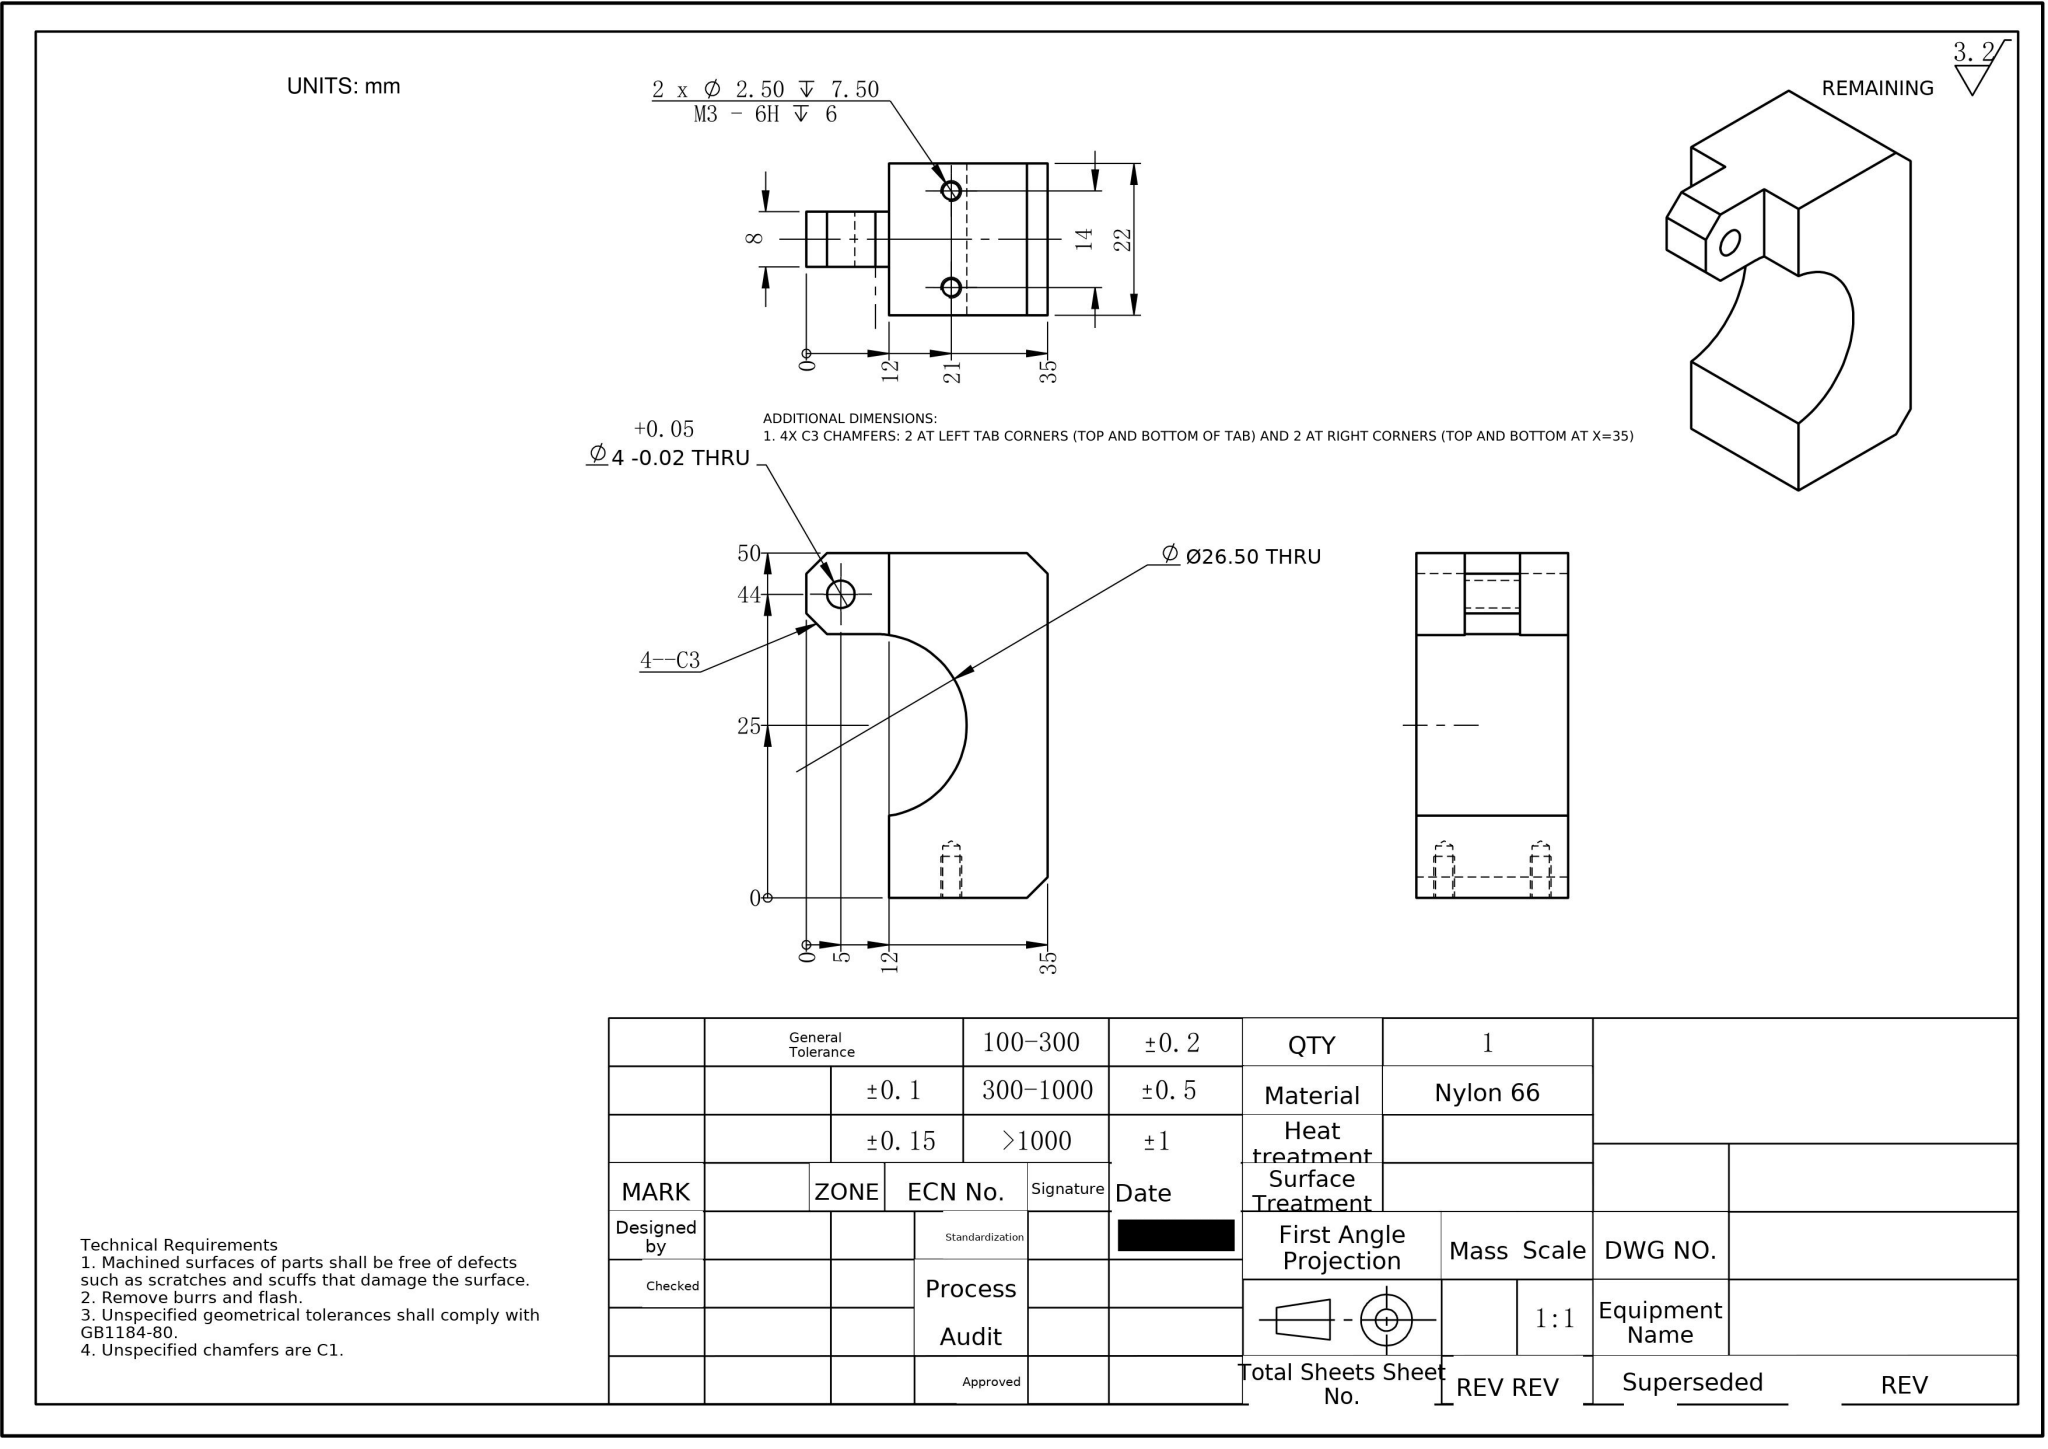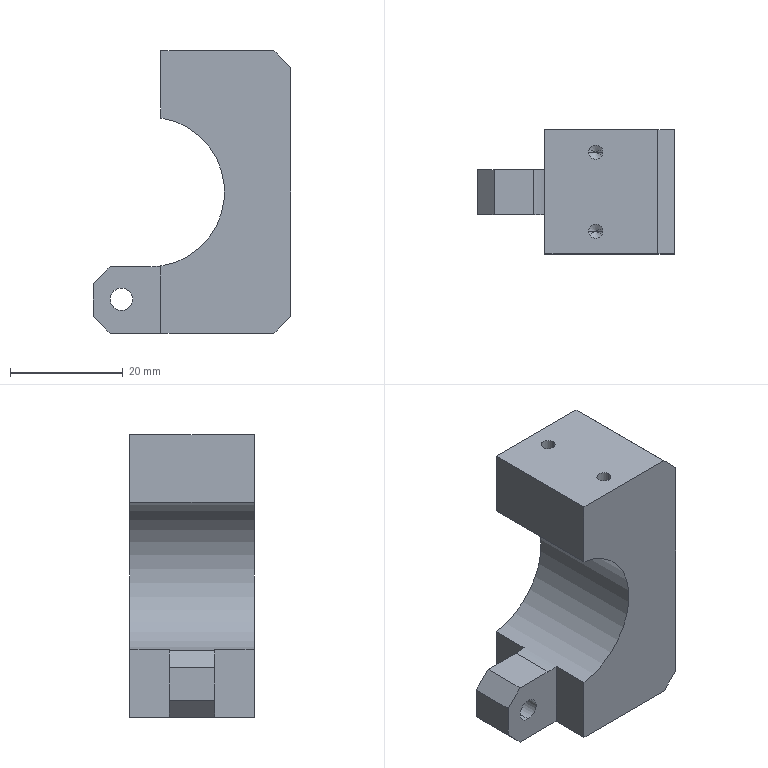Part | NX | mm | 1 solid | 27 faces | box 35 x 22 x 50 mm | volume 21077 mm3 | plane 16 | cylinder 7 | cone 4 | commonest cylinder face diameters 2.5 x4 4 x2 26.5 x1
STEP:
#1=COLOUR_RGB('',0.7922,0.8196,0.9333);
#2=FILL_AREA_STYLE_COLOUR('',#1);
#3=FILL_AREA_STYLE('',(#2));
#4=SURFACE_STYLE_FILL_AREA(#3);
#5=SURFACE_SIDE_STYLE('',(#4));
#6=SURFACE_STYLE_USAGE(.BOTH.,#5);
#7=PRESENTATION_STYLE_ASSIGNMENT((#6));
#8=CARTESIAN_POINT('',(-2.75,-7.,17.5));
#9=VERTEX_POINT('',#8);
#10=CARTESIAN_POINT('',(-0.25,-7.,17.5));
#11=VERTEX_POINT('',#10);
#12=CARTESIAN_POINT('',(-1.5,-7.,17.5));
#13=DIRECTION('',(0.,0.,1.));
#14=DIRECTION('',(1.,0.,0.));
#15=AXIS2_PLACEMENT_3D('',#12,#13,#14);
#16=CIRCLE('',#15,1.25);
#17=EDGE_CURVE('',#9,#11,#16,.T.);
#18=ORIENTED_EDGE('',*,*,#17,.F.);
#19=CARTESIAN_POINT('',(-2.75,-7.,25.));
#20=VERTEX_POINT('',#19);
#21=CARTESIAN_POINT('',(-2.75,-7.,25.));
#22=DIRECTION('',(0.,0.,1.));
#23=VECTOR('',#22,1000.);
#24=LINE('',#21,#23);
#25=EDGE_CURVE('',#9,#20,#24,.T.);
#26=ORIENTED_EDGE('',*,*,#25,.T.);
#27=CARTESIAN_POINT('',(-0.25,-7.,25.));
#28=VERTEX_POINT('',#27);
#29=CARTESIAN_POINT('',(-1.5,-7.,25.));
#30=DIRECTION('',(0.,0.,1.));
#31=DIRECTION('',(1.,0.,0.));
#32=AXIS2_PLACEMENT_3D('',#29,#30,#31);
#33=CIRCLE('',#32,1.25);
#34=EDGE_CURVE('',#20,#28,#33,.T.);
#35=ORIENTED_EDGE('',*,*,#34,.T.);
#36=CARTESIAN_POINT('',(-0.25,-7.,25.));
#37=DIRECTION('',(0.,0.,1.));
#38=VECTOR('',#37,1000.);
#39=LINE('',#36,#38);
#40=EDGE_CURVE('',#11,#28,#39,.T.);
#41=ORIENTED_EDGE('',*,*,#40,.F.);
#42=EDGE_LOOP('',(#18,#26,#35,#41));
#43=FACE_OUTER_BOUND('',#42,.T.);
#44=CARTESIAN_POINT('',(-1.5,-7.,25.));
#45=DIRECTION('',(0.,0.,1.));
#46=DIRECTION('',(1.,0.,0.));
#47=AXIS2_PLACEMENT_3D('',#44,#45,#46);
#48=CYLINDRICAL_SURFACE('',#47,1.25);
#49=ADVANCED_FACE('',(#43),#48,.F.);
#50=CARTESIAN_POINT('',(-1.5,-7.,16.749));
#51=VERTEX_POINT('',#50);
#52=CARTESIAN_POINT('',(-0.25,-7.,17.5));
#53=DIRECTION('',(0.8572,0.,0.515));
#54=VECTOR('',#53,1000.);
#55=LINE('',#52,#54);
#56=EDGE_CURVE('',#51,#11,#55,.T.);
#57=ORIENTED_EDGE('',*,*,#56,.F.);
#58=CARTESIAN_POINT('',(-2.75,-7.,17.5));
#59=DIRECTION('',(-0.8572,0.,0.515));
#60=VECTOR('',#59,1000.);
#61=LINE('',#58,#60);
#62=EDGE_CURVE('',#51,#9,#61,.T.);
#63=ORIENTED_EDGE('',*,*,#62,.T.);
#64=ORIENTED_EDGE('',*,*,#17,.T.);
#65=EDGE_LOOP('',(#57,#63,#64));
#66=FACE_OUTER_BOUND('',#65,.T.);
#67=CARTESIAN_POINT('',(-1.5,-7.,17.5));
#68=DIRECTION('',(0.,0.,1.));
#69=DIRECTION('',(1.,0.,0.));
#70=AXIS2_PLACEMENT_3D('',#67,#68,#69);
#71=CONICAL_SURFACE('',#70,1.25,1.03);
#72=ADVANCED_FACE('',(#66),#71,.F.);
#73=CARTESIAN_POINT('',(-2.75,7.,17.5));
#74=VERTEX_POINT('',#73);
#75=CARTESIAN_POINT('',(-0.25,7.,17.5));
#76=VERTEX_POINT('',#75);
#77=CARTESIAN_POINT('',(-1.5,7.,17.5));
#78=DIRECTION('',(0.,0.,1.));
#79=DIRECTION('',(1.,0.,0.));
#80=AXIS2_PLACEMENT_3D('',#77,#78,#79);
#81=CIRCLE('',#80,1.25);
#82=EDGE_CURVE('',#74,#76,#81,.T.);
#83=ORIENTED_EDGE('',*,*,#82,.F.);
#84=CARTESIAN_POINT('',(-2.75,7.,25.));
#85=VERTEX_POINT('',#84);
#86=CARTESIAN_POINT('',(-2.75,7.,25.));
#87=DIRECTION('',(0.,0.,1.));
#88=VECTOR('',#87,1000.);
#89=LINE('',#86,#88);
#90=EDGE_CURVE('',#74,#85,#89,.T.);
#91=ORIENTED_EDGE('',*,*,#90,.T.);
#92=CARTESIAN_POINT('',(-0.25,7.,25.));
#93=VERTEX_POINT('',#92);
#94=CARTESIAN_POINT('',(-1.5,7.,25.));
#95=DIRECTION('',(0.,0.,1.));
#96=DIRECTION('',(1.,0.,0.));
#97=AXIS2_PLACEMENT_3D('',#94,#95,#96);
#98=CIRCLE('',#97,1.25);
#99=EDGE_CURVE('',#85,#93,#98,.T.);
#100=ORIENTED_EDGE('',*,*,#99,.T.);
#101=CARTESIAN_POINT('',(-0.25,7.,25.));
#102=DIRECTION('',(0.,0.,1.));
#103=VECTOR('',#102,1000.);
#104=LINE('',#101,#103);
#105=EDGE_CURVE('',#76,#93,#104,.T.);
#106=ORIENTED_EDGE('',*,*,#105,.F.);
#107=EDGE_LOOP('',(#83,#91,#100,#106));
#108=FACE_OUTER_BOUND('',#107,.T.);
#109=CARTESIAN_POINT('',(-1.5,7.,25.));
#110=DIRECTION('',(0.,0.,1.));
#111=DIRECTION('',(1.,0.,0.));
#112=AXIS2_PLACEMENT_3D('',#109,#110,#111);
#113=CYLINDRICAL_SURFACE('',#112,1.25);
#114=ADVANCED_FACE('',(#108),#113,.F.);
#115=CARTESIAN_POINT('',(-1.5,7.,16.749));
#116=VERTEX_POINT('',#115);
#117=CARTESIAN_POINT('',(-0.25,7.,17.5));
#118=DIRECTION('',(0.8572,0.,0.515));
#119=VECTOR('',#118,1000.);
#120=LINE('',#117,#119);
#121=EDGE_CURVE('',#116,#76,#120,.T.);
#122=ORIENTED_EDGE('',*,*,#121,.F.);
#123=CARTESIAN_POINT('',(-2.75,7.,17.5));
#124=DIRECTION('',(-0.8572,0.,0.515));
#125=VECTOR('',#124,1000.);
#126=LINE('',#123,#125);
#127=EDGE_CURVE('',#116,#74,#126,.T.);
#128=ORIENTED_EDGE('',*,*,#127,.T.);
#129=ORIENTED_EDGE('',*,*,#82,.T.);
#130=EDGE_LOOP('',(#122,#128,#129));
#131=FACE_OUTER_BOUND('',#130,.T.);
#132=CARTESIAN_POINT('',(-1.5,7.,17.5));
#133=DIRECTION('',(0.,0.,1.));
#134=DIRECTION('',(1.,0.,0.));
#135=AXIS2_PLACEMENT_3D('',#132,#133,#134);
#136=CONICAL_SURFACE('',#135,1.25,1.03);
#137=ADVANCED_FACE('',(#131),#136,.F.);
#138=CARTESIAN_POINT('',(-17.5,4.,-17.));
#139=VERTEX_POINT('',#138);
#140=CARTESIAN_POINT('',(-17.5,4.,-21.));
#141=VERTEX_POINT('',#140);
#142=CARTESIAN_POINT('',(-17.5,4.,-19.));
#143=DIRECTION('',(0.,-1.,0.));
#144=DIRECTION('',(0.,0.,-1.));
#145=AXIS2_PLACEMENT_3D('',#142,#143,#144);
#146=CIRCLE('',#145,2.);
#147=EDGE_CURVE('',#139,#141,#146,.T.);
#148=ORIENTED_EDGE('',*,*,#147,.F.);
#149=CARTESIAN_POINT('',(-17.5,-4.,-17.));
#150=VERTEX_POINT('',#149);
#151=CARTESIAN_POINT('',(-17.5,6.,-17.));
#152=DIRECTION('',(0.,-1.,0.));
#153=VECTOR('',#152,1000.);
#154=LINE('',#151,#153);
#155=EDGE_CURVE('',#139,#150,#154,.T.);
#156=ORIENTED_EDGE('',*,*,#155,.T.);
#157=CARTESIAN_POINT('',(-17.5,-4.,-21.));
#158=VERTEX_POINT('',#157);
#159=CARTESIAN_POINT('',(-17.5,-4.,-19.));
#160=DIRECTION('',(0.,-1.,0.));
#161=DIRECTION('',(0.,0.,-1.));
#162=AXIS2_PLACEMENT_3D('',#159,#160,#161);
#163=CIRCLE('',#162,2.);
#164=EDGE_CURVE('',#150,#158,#163,.T.);
#165=ORIENTED_EDGE('',*,*,#164,.T.);
#166=CARTESIAN_POINT('',(-17.5,6.,-21.));
#167=DIRECTION('',(0.,-1.,0.));
#168=VECTOR('',#167,1000.);
#169=LINE('',#166,#168);
#170=EDGE_CURVE('',#141,#158,#169,.T.);
#171=ORIENTED_EDGE('',*,*,#170,.F.);
#172=EDGE_LOOP('',(#148,#156,#165,#171));
#173=FACE_OUTER_BOUND('',#172,.T.);
#174=CARTESIAN_POINT('',(-17.5,6.,-19.));
#175=DIRECTION('',(0.,-1.,0.));
#176=DIRECTION('',(0.,0.,-1.));
#177=AXIS2_PLACEMENT_3D('',#174,#175,#176);
#178=CYLINDRICAL_SURFACE('',#177,2.);
#179=ADVANCED_FACE('',(#173),#178,.F.);
#180=CARTESIAN_POINT('',(12.5,11.,22.));
#181=VERTEX_POINT('',#180);
#182=CARTESIAN_POINT('',(12.5,11.,-22.));
#183=VERTEX_POINT('',#182);
#184=CARTESIAN_POINT('',(12.5,11.,25.));
#185=DIRECTION('',(0.,0.,-1.));
#186=VECTOR('',#185,1000.);
#187=LINE('',#184,#186);
#188=EDGE_CURVE('',#181,#183,#187,.T.);
#189=ORIENTED_EDGE('',*,*,#188,.F.);
#190=CARTESIAN_POINT('',(12.5,-11.,22.));
#191=VERTEX_POINT('',#190);
#192=CARTESIAN_POINT('',(12.5,11.,22.));
#193=DIRECTION('',(0.,-1.,0.));
#194=VECTOR('',#193,1000.);
#195=LINE('',#192,#194);
#196=EDGE_CURVE('',#181,#191,#195,.T.);
#197=ORIENTED_EDGE('',*,*,#196,.T.);
#198=CARTESIAN_POINT('',(12.5,-11.,-22.));
#199=VERTEX_POINT('',#198);
#200=CARTESIAN_POINT('',(12.5,-11.,25.));
#201=DIRECTION('',(0.,0.,-1.));
#202=VECTOR('',#201,1000.);
#203=LINE('',#200,#202);
#204=EDGE_CURVE('',#191,#199,#203,.T.);
#205=ORIENTED_EDGE('',*,*,#204,.T.);
#206=CARTESIAN_POINT('',(12.5,11.,-22.));
#207=DIRECTION('',(0.,1.,0.));
#208=VECTOR('',#207,1000.);
#209=LINE('',#206,#208);
#210=EDGE_CURVE('',#199,#183,#209,.T.);
#211=ORIENTED_EDGE('',*,*,#210,.T.);
#212=EDGE_LOOP('',(#189,#197,#205,#211));
#213=FACE_OUTER_BOUND('',#212,.T.);
#214=CARTESIAN_POINT('',(12.5,11.,25.));
#215=DIRECTION('',(-1.,0.,0.));
#216=DIRECTION('',(0.,0.,1.));
#217=AXIS2_PLACEMENT_3D('',#214,#215,#216);
#218=PLANE('',#217);
#219=ADVANCED_FACE('',(#213),#218,.F.);
#220=CARTESIAN_POINT('',(-10.5,-4.,-25.));
#221=VERTEX_POINT('',#220);
#222=CARTESIAN_POINT('',(-10.5,-11.,-25.));
#223=VERTEX_POINT('',#222);
#224=CARTESIAN_POINT('',(-10.5,-4.,-25.));
#225=DIRECTION('',(0.,-1.,0.));
#226=VECTOR('',#225,1000.);
#227=LINE('',#224,#226);
#228=EDGE_CURVE('',#221,#223,#227,.T.);
#229=ORIENTED_EDGE('',*,*,#228,.F.);
#230=CARTESIAN_POINT('',(-19.5,-4.,-25.));
#231=VERTEX_POINT('',#230);
#232=CARTESIAN_POINT('',(-22.5,-4.,-25.));
#233=DIRECTION('',(1.,0.,0.));
#234=VECTOR('',#233,1000.);
#235=LINE('',#232,#234);
#236=EDGE_CURVE('',#231,#221,#235,.T.);
#237=ORIENTED_EDGE('',*,*,#236,.F.);
#238=CARTESIAN_POINT('',(-19.5,4.,-25.));
#239=VERTEX_POINT('',#238);
#240=CARTESIAN_POINT('',(-19.5,11.,-25.));
#241=DIRECTION('',(0.,1.,0.));
#242=VECTOR('',#241,1000.);
#243=LINE('',#240,#242);
#244=EDGE_CURVE('',#231,#239,#243,.T.);
#245=ORIENTED_EDGE('',*,*,#244,.T.);
#246=CARTESIAN_POINT('',(-10.5,4.,-25.));
#247=VERTEX_POINT('',#246);
#248=CARTESIAN_POINT('',(-22.5,4.,-25.));
#249=DIRECTION('',(1.,0.,0.));
#250=VECTOR('',#249,1000.);
#251=LINE('',#248,#250);
#252=EDGE_CURVE('',#239,#247,#251,.T.);
#253=ORIENTED_EDGE('',*,*,#252,.T.);
#254=CARTESIAN_POINT('',(-10.5,11.,-25.));
#255=VERTEX_POINT('',#254);
#256=CARTESIAN_POINT('',(-10.5,4.,-25.));
#257=DIRECTION('',(0.,-1.,0.));
#258=VECTOR('',#257,1000.);
#259=LINE('',#256,#258);
#260=EDGE_CURVE('',#255,#247,#259,.T.);
#261=ORIENTED_EDGE('',*,*,#260,.F.);
#262=CARTESIAN_POINT('',(9.5,11.,-25.));
#263=VERTEX_POINT('',#262);
#264=CARTESIAN_POINT('',(-12.5,11.,-25.));
#265=DIRECTION('',(-1.,0.,0.));
#266=VECTOR('',#265,1000.);
#267=LINE('',#264,#266);
#268=EDGE_CURVE('',#263,#255,#267,.T.);
#269=ORIENTED_EDGE('',*,*,#268,.F.);
#270=CARTESIAN_POINT('',(9.5,-11.,-25.));
#271=VERTEX_POINT('',#270);
#272=CARTESIAN_POINT('',(9.5,11.,-25.));
#273=DIRECTION('',(0.,-1.,0.));
#274=VECTOR('',#273,1000.);
#275=LINE('',#272,#274);
#276=EDGE_CURVE('',#263,#271,#275,.T.);
#277=ORIENTED_EDGE('',*,*,#276,.T.);
#278=CARTESIAN_POINT('',(-12.5,-11.,-25.));
#279=DIRECTION('',(-1.,0.,0.));
#280=VECTOR('',#279,1000.);
#281=LINE('',#278,#280);
#282=EDGE_CURVE('',#271,#223,#281,.T.);
#283=ORIENTED_EDGE('',*,*,#282,.T.);
#284=EDGE_LOOP('',(#229,#237,#245,#253,#261,#269,#277,#283));
#285=FACE_OUTER_BOUND('',#284,.T.);
#286=CARTESIAN_POINT('',(-12.5,11.,-25.));
#287=DIRECTION('',(0.,0.,1.));
#288=DIRECTION('',(1.,0.,0.));
#289=AXIS2_PLACEMENT_3D('',#286,#287,#288);
#290=PLANE('',#289);
#291=ADVANCED_FACE('',(#285),#290,.F.);
#292=CARTESIAN_POINT('',(-1.5,-7.,25.));
#293=DIRECTION('',(0.,0.,1.));
#294=DIRECTION('',(1.,0.,0.));
#295=AXIS2_PLACEMENT_3D('',#292,#293,#294);
#296=CIRCLE('',#295,1.25);
#297=EDGE_CURVE('',#28,#20,#296,.T.);
#298=ORIENTED_EDGE('',*,*,#297,.F.);
#299=ORIENTED_EDGE('',*,*,#34,.F.);
#300=EDGE_LOOP('',(#298,#299));
#301=FACE_BOUND('',#300,.T.);
#302=CARTESIAN_POINT('',(-1.5,7.,25.));
#303=DIRECTION('',(0.,0.,1.));
#304=DIRECTION('',(1.,0.,0.));
#305=AXIS2_PLACEMENT_3D('',#302,#303,#304);
#306=CIRCLE('',#305,1.25);
#307=EDGE_CURVE('',#93,#85,#306,.T.);
#308=ORIENTED_EDGE('',*,*,#307,.F.);
#309=ORIENTED_EDGE('',*,*,#99,.F.);
#310=EDGE_LOOP('',(#308,#309));
#311=FACE_BOUND('',#310,.T.);
#312=CARTESIAN_POINT('',(-10.5,11.,25.));
#313=VERTEX_POINT('',#312);
#314=CARTESIAN_POINT('',(9.5,11.,25.));
#315=VERTEX_POINT('',#314);
#316=CARTESIAN_POINT('',(-12.5,11.,25.));
#317=DIRECTION('',(1.,0.,0.));
#318=VECTOR('',#317,1000.);
#319=LINE('',#316,#318);
#320=EDGE_CURVE('',#313,#315,#319,.T.);
#321=ORIENTED_EDGE('',*,*,#320,.F.);
#322=CARTESIAN_POINT('',(-10.5,-11.,25.));
#323=VERTEX_POINT('',#322);
#324=CARTESIAN_POINT('',(-10.5,39.,25.));
#325=DIRECTION('',(0.,-1.,0.));
#326=VECTOR('',#325,1000.);
#327=LINE('',#324,#326);
#328=EDGE_CURVE('',#313,#323,#327,.T.);
#329=ORIENTED_EDGE('',*,*,#328,.T.);
#330=CARTESIAN_POINT('',(9.5,-11.,25.));
#331=VERTEX_POINT('',#330);
#332=CARTESIAN_POINT('',(-12.5,-11.,25.));
#333=DIRECTION('',(1.,0.,0.));
#334=VECTOR('',#333,1000.);
#335=LINE('',#332,#334);
#336=EDGE_CURVE('',#323,#331,#335,.T.);
#337=ORIENTED_EDGE('',*,*,#336,.T.);
#338=CARTESIAN_POINT('',(9.5,11.,25.));
#339=DIRECTION('',(0.,1.,0.));
#340=VECTOR('',#339,1000.);
#341=LINE('',#338,#340);
#342=EDGE_CURVE('',#331,#315,#341,.T.);
#343=ORIENTED_EDGE('',*,*,#342,.T.);
#344=EDGE_LOOP('',(#321,#329,#337,#343));
#345=FACE_OUTER_BOUND('',#344,.T.);
#346=CARTESIAN_POINT('',(-12.5,11.,25.));
#347=DIRECTION('',(0.,0.,-1.));
#348=DIRECTION('',(-1.,0.,0.));
#349=AXIS2_PLACEMENT_3D('',#346,#347,#348);
#350=PLANE('',#349);
#351=ADVANCED_FACE('',(#301,#311,#345),#350,.F.);
#352=ORIENTED_EDGE('',*,*,#268,.T.);
#353=CARTESIAN_POINT('',(-10.5,11.,-13.098));
#354=VERTEX_POINT('',#353);
#355=CARTESIAN_POINT('',(-10.5,11.,-5.));
#356=DIRECTION('',(0.,0.,-1.));
#357=VECTOR('',#356,1000.);
#358=LINE('',#355,#357);
#359=EDGE_CURVE('',#354,#255,#358,.T.);
#360=ORIENTED_EDGE('',*,*,#359,.F.);
#361=CARTESIAN_POINT('',(-10.5,11.,13.098));
#362=VERTEX_POINT('',#361);
#363=CARTESIAN_POINT('',(-12.5,11.,0.));
#364=DIRECTION('',(0.,-1.,0.));
#365=DIRECTION('',(0.,0.,-1.));
#366=AXIS2_PLACEMENT_3D('',#363,#364,#365);
#367=CIRCLE('',#366,13.25);
#368=EDGE_CURVE('',#354,#362,#367,.T.);
#369=ORIENTED_EDGE('',*,*,#368,.T.);
#370=CARTESIAN_POINT('',(-10.5,11.,-0.));
#371=DIRECTION('',(-0.,0.,1.));
#372=VECTOR('',#371,1000.);
#373=LINE('',#370,#372);
#374=EDGE_CURVE('',#362,#313,#373,.T.);
#375=ORIENTED_EDGE('',*,*,#374,.T.);
#376=ORIENTED_EDGE('',*,*,#320,.T.);
#377=CARTESIAN_POINT('',(12.5,11.,22.));
#378=DIRECTION('',(0.7071,0.,-0.7071));
#379=VECTOR('',#378,1000.);
#380=LINE('',#377,#379);
#381=EDGE_CURVE('',#315,#181,#380,.T.);
#382=ORIENTED_EDGE('',*,*,#381,.T.);
#383=ORIENTED_EDGE('',*,*,#188,.T.);
#384=CARTESIAN_POINT('',(9.5,11.,-25.));
#385=DIRECTION('',(-0.7071,0.,-0.7071));
#386=VECTOR('',#385,1000.);
#387=LINE('',#384,#386);
#388=EDGE_CURVE('',#183,#263,#387,.T.);
#389=ORIENTED_EDGE('',*,*,#388,.T.);
#390=EDGE_LOOP('',(#352,#360,#369,#375,#376,#382,#383,#389));
#391=FACE_OUTER_BOUND('',#390,.T.);
#392=CARTESIAN_POINT('',(0.,11.,0.));
#393=DIRECTION('',(0.,-1.,0.));
#394=DIRECTION('',(0.,0.,-1.));
#395=AXIS2_PLACEMENT_3D('',#392,#393,#394);
#396=PLANE('',#395);
#397=ADVANCED_FACE('',(#391),#396,.F.);
#398=CARTESIAN_POINT('',(-10.5,-11.,-13.098));
#399=VERTEX_POINT('',#398);
#400=CARTESIAN_POINT('',(-10.5,-11.,-5.));
#401=DIRECTION('',(0.,0.,-1.));
#402=VECTOR('',#401,1000.);
#403=LINE('',#400,#402);
#404=EDGE_CURVE('',#399,#223,#403,.T.);
#405=ORIENTED_EDGE('',*,*,#404,.T.);
#406=ORIENTED_EDGE('',*,*,#282,.F.);
#407=CARTESIAN_POINT('',(17.25,-11.,-17.25));
#408=DIRECTION('',(0.7071,0.,0.7071));
#409=VECTOR('',#408,1000.);
#410=LINE('',#407,#409);
#411=EDGE_CURVE('',#271,#199,#410,.T.);
#412=ORIENTED_EDGE('',*,*,#411,.T.);
#413=ORIENTED_EDGE('',*,*,#204,.F.);
#414=CARTESIAN_POINT('',(17.25,-11.,17.25));
#415=DIRECTION('',(-0.7071,0.,0.7071));
#416=VECTOR('',#415,1000.);
#417=LINE('',#414,#416);
#418=EDGE_CURVE('',#191,#331,#417,.T.);
#419=ORIENTED_EDGE('',*,*,#418,.T.);
#420=ORIENTED_EDGE('',*,*,#336,.F.);
#421=CARTESIAN_POINT('',(-10.5,-11.,13.098));
#422=VERTEX_POINT('',#421);
#423=CARTESIAN_POINT('',(-10.5,-11.,25.));
#424=DIRECTION('',(-0.,0.,1.));
#425=VECTOR('',#424,1000.);
#426=LINE('',#423,#425);
#427=EDGE_CURVE('',#422,#323,#426,.T.);
#428=ORIENTED_EDGE('',*,*,#427,.F.);
#429=CARTESIAN_POINT('',(-12.5,-11.,0.));
#430=DIRECTION('',(0.,-1.,0.));
#431=DIRECTION('',(0.,0.,-1.));
#432=AXIS2_PLACEMENT_3D('',#429,#430,#431);
#433=CIRCLE('',#432,13.25);
#434=EDGE_CURVE('',#399,#422,#433,.T.);
#435=ORIENTED_EDGE('',*,*,#434,.F.);
#436=EDGE_LOOP('',(#405,#406,#412,#413,#419,#420,#428,#435));
#437=FACE_OUTER_BOUND('',#436,.T.);
#438=CARTESIAN_POINT('',(0.,-11.,0.));
#439=DIRECTION('',(0.,-1.,0.));
#440=DIRECTION('',(0.,0.,-1.));
#441=AXIS2_PLACEMENT_3D('',#438,#439,#440);
#442=PLANE('',#441);
#443=ADVANCED_FACE('',(#437),#442,.T.);
#444=CARTESIAN_POINT('',(-12.5,-4.,-13.25));
#445=VERTEX_POINT('',#444);
#446=CARTESIAN_POINT('',(-12.5,4.,-13.25));
#447=VERTEX_POINT('',#446);
#448=CARTESIAN_POINT('',(-12.5,-4.,-13.25));
#449=DIRECTION('',(0.,1.,0.));
#450=VECTOR('',#449,1000.);
#451=LINE('',#448,#450);
#452=EDGE_CURVE('',#445,#447,#451,.T.);
#453=ORIENTED_EDGE('',*,*,#452,.F.);
#454=CARTESIAN_POINT('',(-10.5,-4.,-13.098));
#455=VERTEX_POINT('',#454);
#456=CARTESIAN_POINT('',(-12.5,-4.,0.));
#457=DIRECTION('',(-0.,-1.,0.));
#458=DIRECTION('',(-1.,0.,0.));
#459=AXIS2_PLACEMENT_3D('',#456,#457,#458);
#460=CIRCLE('',#459,13.25);
#461=EDGE_CURVE('',#445,#455,#460,.T.);
#462=ORIENTED_EDGE('',*,*,#461,.T.);
#463=CARTESIAN_POINT('',(-10.5,21.,-13.098));
#464=DIRECTION('',(0.,-1.,0.));
#465=VECTOR('',#464,1000.);
#466=LINE('',#463,#465);
#467=EDGE_CURVE('',#455,#399,#466,.T.);
#468=ORIENTED_EDGE('',*,*,#467,.T.);
#469=ORIENTED_EDGE('',*,*,#434,.T.);
#470=CARTESIAN_POINT('',(-10.5,21.,13.098));
#471=DIRECTION('',(0.,1.,0.));
#472=VECTOR('',#471,1000.);
#473=LINE('',#470,#472);
#474=EDGE_CURVE('',#422,#362,#473,.T.);
#475=ORIENTED_EDGE('',*,*,#474,.T.);
#476=ORIENTED_EDGE('',*,*,#368,.F.);
#477=CARTESIAN_POINT('',(-10.5,4.,-13.098));
#478=VERTEX_POINT('',#477);
#479=CARTESIAN_POINT('',(-10.5,21.,-13.098));
#480=DIRECTION('',(0.,-1.,0.));
#481=VECTOR('',#480,1000.);
#482=LINE('',#479,#481);
#483=EDGE_CURVE('',#354,#478,#482,.T.);
#484=ORIENTED_EDGE('',*,*,#483,.T.);
#485=CARTESIAN_POINT('',(-12.5,4.,0.));
#486=DIRECTION('',(-0.,1.,0.));
#487=DIRECTION('',(1.,0.,0.));
#488=AXIS2_PLACEMENT_3D('',#485,#486,#487);
#489=CIRCLE('',#488,13.25);
#490=EDGE_CURVE('',#478,#447,#489,.T.);
#491=ORIENTED_EDGE('',*,*,#490,.T.);
#492=EDGE_LOOP('',(#453,#462,#468,#469,#475,#476,#484,#491));
#493=FACE_OUTER_BOUND('',#492,.T.);
#494=CARTESIAN_POINT('',(-12.5,21.,0.));
#495=DIRECTION('',(0.,-1.,0.));
#496=DIRECTION('',(0.,0.,-1.));
#497=AXIS2_PLACEMENT_3D('',#494,#495,#496);
#498=CYLINDRICAL_SURFACE('',#497,13.25);
#499=ADVANCED_FACE('',(#493),#498,.F.);
#500=ORIENTED_EDGE('',*,*,#381,.F.);
#501=ORIENTED_EDGE('',*,*,#342,.F.);
#502=ORIENTED_EDGE('',*,*,#418,.F.);
#503=ORIENTED_EDGE('',*,*,#196,.F.);
#504=EDGE_LOOP('',(#500,#501,#502,#503));
#505=FACE_OUTER_BOUND('',#504,.T.);
#506=CARTESIAN_POINT('',(12.5,11.,22.));
#507=DIRECTION('',(-0.7071,0.,-0.7071));
#508=DIRECTION('',(0.,-1.,0.));
#509=AXIS2_PLACEMENT_3D('',#506,#507,#508);
#510=PLANE('',#509);
#511=ADVANCED_FACE('',(#505),#510,.F.);
#512=ORIENTED_EDGE('',*,*,#388,.F.);
#513=ORIENTED_EDGE('',*,*,#210,.F.);
#514=ORIENTED_EDGE('',*,*,#411,.F.);
#515=ORIENTED_EDGE('',*,*,#276,.F.);
#516=EDGE_LOOP('',(#512,#513,#514,#515));
#517=FACE_OUTER_BOUND('',#516,.T.);
#518=CARTESIAN_POINT('',(9.5,11.,-25.));
#519=DIRECTION('',(-0.7071,0.,0.7071));
#520=DIRECTION('',(0.,-1.,0.));
#521=AXIS2_PLACEMENT_3D('',#518,#519,#520);
#522=PLANE('',#521);
#523=ADVANCED_FACE('',(#517),#522,.F.);
#524=CARTESIAN_POINT('',(-19.5,4.,-13.25));
#525=VERTEX_POINT('',#524);
#526=CARTESIAN_POINT('',(-22.5,4.,-13.25));
#527=DIRECTION('',(1.,0.,0.));
#528=VECTOR('',#527,1000.);
#529=LINE('',#526,#528);
#530=EDGE_CURVE('',#525,#447,#529,.T.);
#531=ORIENTED_EDGE('',*,*,#530,.F.);
#532=CARTESIAN_POINT('',(-19.5,-4.,-13.25));
#533=VERTEX_POINT('',#532);
#534=CARTESIAN_POINT('',(-19.5,-4.,-13.25));
#535=DIRECTION('',(0.,-1.,0.));
#536=VECTOR('',#535,1000.);
#537=LINE('',#534,#536);
#538=EDGE_CURVE('',#525,#533,#537,.T.);
#539=ORIENTED_EDGE('',*,*,#538,.T.);
#540=CARTESIAN_POINT('',(-22.5,-4.,-13.25));
#541=DIRECTION('',(1.,0.,0.));
#542=VECTOR('',#541,1000.);
#543=LINE('',#540,#542);
#544=EDGE_CURVE('',#533,#445,#543,.T.);
#545=ORIENTED_EDGE('',*,*,#544,.T.);
#546=ORIENTED_EDGE('',*,*,#452,.T.);
#547=EDGE_LOOP('',(#531,#539,#545,#546));
#548=FACE_OUTER_BOUND('',#547,.T.);
#549=CARTESIAN_POINT('',(-22.5,-4.,-13.25));
#550=DIRECTION('',(0.,0.,-1.));
#551=DIRECTION('',(-1.,0.,0.));
#552=AXIS2_PLACEMENT_3D('',#549,#550,#551);
#553=PLANE('',#552);
#554=ADVANCED_FACE('',(#548),#553,.F.);
#555=CARTESIAN_POINT('',(-17.5,4.,-19.));
#556=DIRECTION('',(0.,-1.,0.));
#557=DIRECTION('',(0.,0.,-1.));
#558=AXIS2_PLACEMENT_3D('',#555,#556,#557);
#559=CIRCLE('',#558,2.);
#560=EDGE_CURVE('',#141,#139,#559,.T.);
#561=ORIENTED_EDGE('',*,*,#560,.T.);
#562=ORIENTED_EDGE('',*,*,#147,.T.);
#563=EDGE_LOOP('',(#561,#562));
#564=FACE_BOUND('',#563,.T.);
#565=ORIENTED_EDGE('',*,*,#252,.F.);
#566=CARTESIAN_POINT('',(-22.5,4.,-22.));
#567=VERTEX_POINT('',#566);
#568=CARTESIAN_POINT('',(-22.5,4.,-22.));
#569=DIRECTION('',(-0.7071,0.,0.7071));
#570=VECTOR('',#569,1000.);
#571=LINE('',#568,#570);
#572=EDGE_CURVE('',#239,#567,#571,.T.);
#573=ORIENTED_EDGE('',*,*,#572,.T.);
#574=CARTESIAN_POINT('',(-22.5,4.,-16.25));
#575=VERTEX_POINT('',#574);
#576=CARTESIAN_POINT('',(-22.5,4.,-25.));
#577=DIRECTION('',(0.,0.,-1.));
#578=VECTOR('',#577,1000.);
#579=LINE('',#576,#578);
#580=EDGE_CURVE('',#575,#567,#579,.T.);
#581=ORIENTED_EDGE('',*,*,#580,.F.);
#582=CARTESIAN_POINT('',(-22.5,4.,-16.25));
#583=DIRECTION('',(0.7071,0.,0.7071));
#584=VECTOR('',#583,1000.);
#585=LINE('',#582,#584);
#586=EDGE_CURVE('',#575,#525,#585,.T.);
#587=ORIENTED_EDGE('',*,*,#586,.T.);
#588=ORIENTED_EDGE('',*,*,#530,.T.);
#589=ORIENTED_EDGE('',*,*,#490,.F.);
#590=CARTESIAN_POINT('',(-10.5,4.,-5.));
#591=DIRECTION('',(0.,0.,-1.));
#592=VECTOR('',#591,1000.);
#593=LINE('',#590,#592);
#594=EDGE_CURVE('',#478,#247,#593,.T.);
#595=ORIENTED_EDGE('',*,*,#594,.T.);
#596=EDGE_LOOP('',(#565,#573,#581,#587,#588,#589,#595));
#597=FACE_OUTER_BOUND('',#596,.T.);
#598=CARTESIAN_POINT('',(-22.5,4.,-25.));
#599=DIRECTION('',(0.,-1.,0.));
#600=DIRECTION('',(0.,0.,-1.));
#601=AXIS2_PLACEMENT_3D('',#598,#599,#600);
#602=PLANE('',#601);
#603=ADVANCED_FACE('',(#564,#597),#602,.F.);
#604=CARTESIAN_POINT('',(-17.5,-4.,-19.));
#605=DIRECTION('',(0.,-1.,0.));
#606=DIRECTION('',(0.,0.,-1.));
#607=AXIS2_PLACEMENT_3D('',#604,#605,#606);
#608=CIRCLE('',#607,2.);
#609=EDGE_CURVE('',#158,#150,#608,.T.);
#610=ORIENTED_EDGE('',*,*,#609,.F.);
#611=ORIENTED_EDGE('',*,*,#164,.F.);
#612=EDGE_LOOP('',(#610,#611));
#613=FACE_BOUND('',#612,.T.);
#614=CARTESIAN_POINT('',(-22.5,-4.,-22.));
#615=VERTEX_POINT('',#614);
#616=CARTESIAN_POINT('',(-22.5,-4.,-16.25));
#617=VERTEX_POINT('',#616);
#618=CARTESIAN_POINT('',(-22.5,-4.,-25.));
#619=DIRECTION('',(0.,0.,1.));
#620=VECTOR('',#619,1000.);
#621=LINE('',#618,#620);
#622=EDGE_CURVE('',#615,#617,#621,.T.);
#623=ORIENTED_EDGE('',*,*,#622,.F.);
#624=CARTESIAN_POINT('',(-22.5,-4.,-22.));
#625=DIRECTION('',(0.7071,0.,-0.7071));
#626=VECTOR('',#625,1000.);
#627=LINE('',#624,#626);
#628=EDGE_CURVE('',#615,#231,#627,.T.);
#629=ORIENTED_EDGE('',*,*,#628,.T.);
#630=ORIENTED_EDGE('',*,*,#236,.T.);
#631=CARTESIAN_POINT('',(-10.5,-4.,-5.));
#632=DIRECTION('',(0.,0.,-1.));
#633=VECTOR('',#632,1000.);
#634=LINE('',#631,#633);
#635=EDGE_CURVE('',#455,#221,#634,.T.);
#636=ORIENTED_EDGE('',*,*,#635,.F.);
#637=ORIENTED_EDGE('',*,*,#461,.F.);
#638=ORIENTED_EDGE('',*,*,#544,.F.);
#639=CARTESIAN_POINT('',(-22.5,-4.,-16.25));
#640=DIRECTION('',(-0.7071,0.,-0.7071));
#641=VECTOR('',#640,1000.);
#642=LINE('',#639,#641);
#643=EDGE_CURVE('',#533,#617,#642,.T.);
#644=ORIENTED_EDGE('',*,*,#643,.T.);
#645=EDGE_LOOP('',(#623,#629,#630,#636,#637,#638,#644));
#646=FACE_OUTER_BOUND('',#645,.T.);
#647=CARTESIAN_POINT('',(-22.5,-4.,-25.));
#648=DIRECTION('',(0.,1.,0.));
#649=DIRECTION('',(0.,0.,1.));
#650=AXIS2_PLACEMENT_3D('',#647,#648,#649);
#651=PLANE('',#650);
#652=ADVANCED_FACE('',(#613,#646),#651,.F.);
#653=ORIENTED_EDGE('',*,*,#580,.T.);
#654=CARTESIAN_POINT('',(-22.5,0.,-22.));
#655=DIRECTION('',(0.,-1.,0.));
#656=VECTOR('',#655,1000.);
#657=LINE('',#654,#656);
#658=EDGE_CURVE('',#567,#615,#657,.T.);
#659=ORIENTED_EDGE('',*,*,#658,.T.);
#660=ORIENTED_EDGE('',*,*,#622,.T.);
#661=CARTESIAN_POINT('',(-22.5,0.,-16.25));
#662=DIRECTION('',(0.,1.,0.));
#663=VECTOR('',#662,1000.);
#664=LINE('',#661,#663);
#665=EDGE_CURVE('',#617,#575,#664,.T.);
#666=ORIENTED_EDGE('',*,*,#665,.T.);
#667=EDGE_LOOP('',(#653,#659,#660,#666));
#668=FACE_OUTER_BOUND('',#667,.T.);
#669=CARTESIAN_POINT('',(-22.5,0.,0.));
#670=DIRECTION('',(1.,0.,0.));
#671=DIRECTION('',(0.,0.,-1.));
#672=AXIS2_PLACEMENT_3D('',#669,#670,#671);
#673=PLANE('',#672);
#674=ADVANCED_FACE('',(#668),#673,.F.);
#675=ORIENTED_EDGE('',*,*,#572,.F.);
#676=ORIENTED_EDGE('',*,*,#244,.F.);
#677=ORIENTED_EDGE('',*,*,#628,.F.);
#678=ORIENTED_EDGE('',*,*,#658,.F.);
#679=EDGE_LOOP('',(#675,#676,#677,#678));
#680=FACE_OUTER_BOUND('',#679,.T.);
#681=CARTESIAN_POINT('',(-22.5,0.,-22.));
#682=DIRECTION('',(0.7071,0.,0.7071));
#683=DIRECTION('',(0.,-1.,0.));
#684=AXIS2_PLACEMENT_3D('',#681,#682,#683);
#685=PLANE('',#684);
#686=ADVANCED_FACE('',(#680),#685,.F.);
#687=ORIENTED_EDGE('',*,*,#643,.F.);
#688=ORIENTED_EDGE('',*,*,#538,.F.);
#689=ORIENTED_EDGE('',*,*,#586,.F.);
#690=ORIENTED_EDGE('',*,*,#665,.F.);
#691=EDGE_LOOP('',(#687,#688,#689,#690));
#692=FACE_OUTER_BOUND('',#691,.T.);
#693=CARTESIAN_POINT('',(-22.5,0.,-16.25));
#694=DIRECTION('',(0.7071,0.,-0.7071));
#695=DIRECTION('',(0.,1.,0.));
#696=AXIS2_PLACEMENT_3D('',#693,#694,#695);
#697=PLANE('',#696);
#698=ADVANCED_FACE('',(#692),#697,.F.);
#699=ORIENTED_EDGE('',*,*,#155,.F.);
#700=ORIENTED_EDGE('',*,*,#560,.F.);
#701=ORIENTED_EDGE('',*,*,#170,.T.);
#702=ORIENTED_EDGE('',*,*,#609,.T.);
#703=EDGE_LOOP('',(#699,#700,#701,#702));
#704=FACE_OUTER_BOUND('',#703,.T.);
#705=CARTESIAN_POINT('',(-17.5,6.,-19.));
#706=DIRECTION('',(0.,-1.,0.));
#707=DIRECTION('',(0.,0.,-1.));
#708=AXIS2_PLACEMENT_3D('',#705,#706,#707);
#709=CYLINDRICAL_SURFACE('',#708,2.);
#710=ADVANCED_FACE('',(#704),#709,.F.);
#711=ORIENTED_EDGE('',*,*,#474,.F.);
#712=ORIENTED_EDGE('',*,*,#427,.T.);
#713=ORIENTED_EDGE('',*,*,#328,.F.);
#714=ORIENTED_EDGE('',*,*,#374,.F.);
#715=EDGE_LOOP('',(#711,#712,#713,#714));
#716=FACE_OUTER_BOUND('',#715,.T.);
#717=CARTESIAN_POINT('',(-10.5,39.,25.));
#718=DIRECTION('',(1.,0.,0.));
#719=DIRECTION('',(0.,0.,-1.));
#720=AXIS2_PLACEMENT_3D('',#717,#718,#719);
#721=PLANE('',#720);
#722=ADVANCED_FACE('',(#716),#721,.F.);
#723=ORIENTED_EDGE('',*,*,#359,.T.);
#724=ORIENTED_EDGE('',*,*,#260,.T.);
#725=ORIENTED_EDGE('',*,*,#594,.F.);
#726=ORIENTED_EDGE('',*,*,#483,.F.);
#727=EDGE_LOOP('',(#723,#724,#725,#726));
#728=FACE_OUTER_BOUND('',#727,.T.);
#729=CARTESIAN_POINT('',(-10.5,4.,-5.));
#730=DIRECTION('',(1.,0.,0.));
#731=DIRECTION('',(0.,0.,-1.));
#732=AXIS2_PLACEMENT_3D('',#729,#730,#731);
#733=PLANE('',#732);
#734=ADVANCED_FACE('',(#728),#733,.F.);
#735=ORIENTED_EDGE('',*,*,#635,.T.);
#736=ORIENTED_EDGE('',*,*,#228,.T.);
#737=ORIENTED_EDGE('',*,*,#404,.F.);
#738=ORIENTED_EDGE('',*,*,#467,.F.);
#739=EDGE_LOOP('',(#735,#736,#737,#738));
#740=FACE_OUTER_BOUND('',#739,.T.);
#741=CARTESIAN_POINT('',(-10.5,-4.,-5.));
#742=DIRECTION('',(1.,0.,0.));
#743=DIRECTION('',(0.,0.,-1.));
#744=AXIS2_PLACEMENT_3D('',#741,#742,#743);
#745=PLANE('',#744);
#746=ADVANCED_FACE('',(#740),#745,.F.);
#747=ORIENTED_EDGE('',*,*,#127,.F.);
#748=ORIENTED_EDGE('',*,*,#121,.T.);
#749=CARTESIAN_POINT('',(-1.5,7.,17.5));
#750=DIRECTION('',(0.,0.,1.));
#751=DIRECTION('',(1.,0.,0.));
#752=AXIS2_PLACEMENT_3D('',#749,#750,#751);
#753=CIRCLE('',#752,1.25);
#754=EDGE_CURVE('',#76,#74,#753,.T.);
#755=ORIENTED_EDGE('',*,*,#754,.T.);
#756=EDGE_LOOP('',(#747,#748,#755));
#757=FACE_OUTER_BOUND('',#756,.T.);
#758=CARTESIAN_POINT('',(-1.5,7.,17.5));
#759=DIRECTION('',(0.,0.,1.));
#760=DIRECTION('',(1.,0.,0.));
#761=AXIS2_PLACEMENT_3D('',#758,#759,#760);
#762=CONICAL_SURFACE('',#761,1.25,1.03);
#763=ADVANCED_FACE('',(#757),#762,.F.);
#764=ORIENTED_EDGE('',*,*,#90,.F.);
#765=ORIENTED_EDGE('',*,*,#754,.F.);
#766=ORIENTED_EDGE('',*,*,#105,.T.);
#767=ORIENTED_EDGE('',*,*,#307,.T.);
#768=EDGE_LOOP('',(#764,#765,#766,#767));
#769=FACE_OUTER_BOUND('',#768,.T.);
#770=CARTESIAN_POINT('',(-1.5,7.,25.));
#771=DIRECTION('',(0.,0.,1.));
#772=DIRECTION('',(1.,0.,0.));
#773=AXIS2_PLACEMENT_3D('',#770,#771,#772);
#774=CYLINDRICAL_SURFACE('',#773,1.25);
#775=ADVANCED_FACE('',(#769),#774,.F.);
#776=ORIENTED_EDGE('',*,*,#62,.F.);
#777=ORIENTED_EDGE('',*,*,#56,.T.);
#778=CARTESIAN_POINT('',(-1.5,-7.,17.5));
#779=DIRECTION('',(0.,0.,1.));
#780=DIRECTION('',(1.,0.,0.));
#781=AXIS2_PLACEMENT_3D('',#778,#779,#780);
#782=CIRCLE('',#781,1.25);
#783=EDGE_CURVE('',#11,#9,#782,.T.);
#784=ORIENTED_EDGE('',*,*,#783,.T.);
#785=EDGE_LOOP('',(#776,#777,#784));
#786=FACE_OUTER_BOUND('',#785,.T.);
#787=CARTESIAN_POINT('',(-1.5,-7.,17.5));
#788=DIRECTION('',(0.,0.,1.));
#789=DIRECTION('',(1.,0.,0.));
#790=AXIS2_PLACEMENT_3D('',#787,#788,#789);
#791=CONICAL_SURFACE('',#790,1.25,1.03);
#792=ADVANCED_FACE('',(#786),#791,.F.);
#793=ORIENTED_EDGE('',*,*,#25,.F.);
#794=ORIENTED_EDGE('',*,*,#783,.F.);
#795=ORIENTED_EDGE('',*,*,#40,.T.);
#796=ORIENTED_EDGE('',*,*,#297,.T.);
#797=EDGE_LOOP('',(#793,#794,#795,#796));
#798=FACE_OUTER_BOUND('',#797,.T.);
#799=CARTESIAN_POINT('',(-1.5,-7.,25.));
#800=DIRECTION('',(0.,0.,1.));
#801=DIRECTION('',(1.,0.,0.));
#802=AXIS2_PLACEMENT_3D('',#799,#800,#801);
#803=CYLINDRICAL_SURFACE('',#802,1.25);
#804=ADVANCED_FACE('',(#798),#803,.F.);
#805=CLOSED_SHELL('',(#49,#72,#114,#137,#179,#219,#291,#351,#397,#443,#499,#511,#523,#554,#603,#652,#674,#686,#698,#710,#722,#734,#746,#763,#775,#792,#804));
#806=MANIFOLD_SOLID_BREP('',#805);
#807=STYLED_ITEM('',(#7),#806);
#808=(LENGTH_UNIT()NAMED_UNIT(*)SI_UNIT(.MILLI.,.METRE.));
#809=UNCERTAINTY_MEASURE_WITH_UNIT(LENGTH_MEASURE(0.00001),#808,'','');
#810=(NAMED_UNIT(*)PLANE_ANGLE_UNIT()SI_UNIT($,.RADIAN.));
#811=(NAMED_UNIT(*)SI_UNIT($,.STERADIAN.)SOLID_ANGLE_UNIT());
#812=(GEOMETRIC_REPRESENTATION_CONTEXT(3)GLOBAL_UNCERTAINTY_ASSIGNED_CONTEXT((#809))GLOBAL_UNIT_ASSIGNED_CONTEXT((#808,#810,#811))REPRESENTATION_CONTEXT('',''));
#813=MECHANICAL_DESIGN_GEOMETRIC_PRESENTATION_REPRESENTATION('',(#807),#812);
#814=PRESENTATION_LAYER_ASSIGNMENT('','',(#807));
#815=CARTESIAN_POINT('',(0.,0.,0.));
#816=DIRECTION('',(0.,0.,1.));
#817=DIRECTION('',(1.,0.,0.));
#818=AXIS2_PLACEMENT_3D('',#815,#816,#817);
#819=(LENGTH_UNIT()NAMED_UNIT(*)SI_UNIT(.MILLI.,.METRE.));
#820=UNCERTAINTY_MEASURE_WITH_UNIT(LENGTH_MEASURE(0.00001),#819,'','');
#821=(NAMED_UNIT(*)PLANE_ANGLE_UNIT()SI_UNIT($,.RADIAN.));
#822=(NAMED_UNIT(*)SI_UNIT($,.STERADIAN.)SOLID_ANGLE_UNIT());
#823=(GEOMETRIC_REPRESENTATION_CONTEXT(3)GLOBAL_UNCERTAINTY_ASSIGNED_CONTEXT((#820))GLOBAL_UNIT_ASSIGNED_CONTEXT((#819,#821,#822))REPRESENTATION_CONTEXT('',''));
#824=ADVANCED_BREP_SHAPE_REPRESENTATION('',(#806,#818),#823);